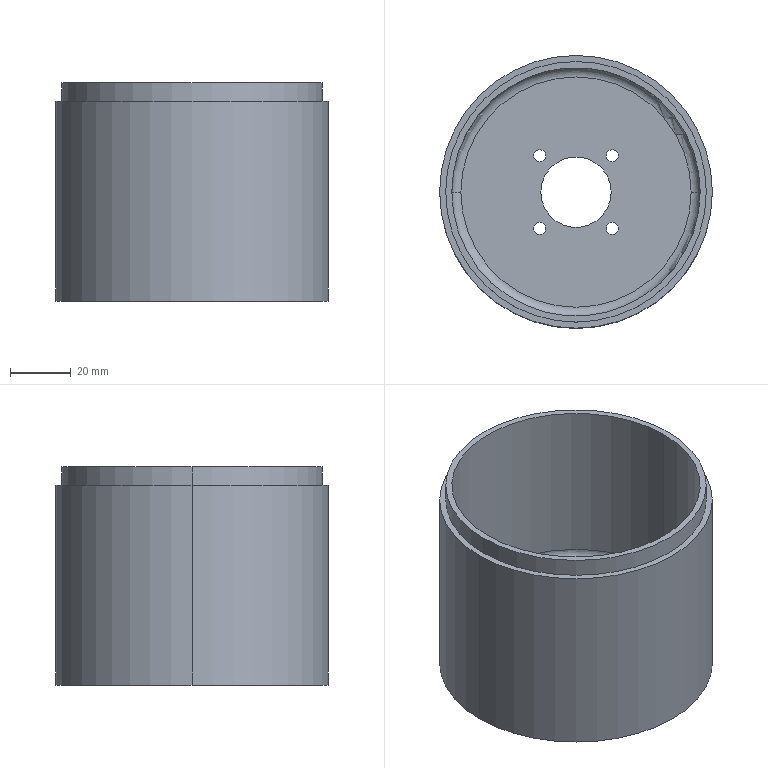Component | SolidWorks | g11-1 | 1 solid | 29 faces | box 90 x 90 x 72 mm | volume 87724 mm3 | cylinder 18 | plane 6 | torus 4 | sphere 1 | commonest cylinder face diameters 4 x8 86 x4 82 x4 90 x2
STEP:
#1=COLOUR_RGB('',0.7922,0.8196,0.9333);
#2=FILL_AREA_STYLE_COLOUR('',#1);
#3=FILL_AREA_STYLE('',(#2));
#4=SURFACE_STYLE_FILL_AREA(#3);
#5=SURFACE_SIDE_STYLE('',(#4));
#6=SURFACE_STYLE_USAGE(.BOTH.,#5);
#7=PRESENTATION_STYLE_ASSIGNMENT((#6));
#8=CARTESIAN_POINT('',(1.066,-0.06694,2.598));
#9=VERTEX_POINT('',#8);
#10=CARTESIAN_POINT('',(-2.32,-0.06694,2.598));
#11=VERTEX_POINT('',#10);
#12=CARTESIAN_POINT('',(-0.6271,-0.06694,2.598));
#13=DIRECTION('',(0.,0.,-1.));
#14=DIRECTION('',(-1.,0.,0.));
#15=AXIS2_PLACEMENT_3D('',#12,#13,#14);
#16=CIRCLE('',#15,1.693);
#17=EDGE_CURVE('',#9,#11,#16,.T.);
#18=ORIENTED_EDGE('',*,*,#17,.F.);
#19=CARTESIAN_POINT('',(1.066,-0.06694,2.441));
#20=VERTEX_POINT('',#19);
#21=CARTESIAN_POINT('',(1.066,-0.06694,2.165));
#22=DIRECTION('',(0.,0.,-1.));
#23=VECTOR('',#22,39.37);
#24=LINE('',#21,#23);
#25=EDGE_CURVE('',#9,#20,#24,.T.);
#26=ORIENTED_EDGE('',*,*,#25,.T.);
#27=CARTESIAN_POINT('',(-2.32,-0.06694,2.441));
#28=VERTEX_POINT('',#27);
#29=CARTESIAN_POINT('',(-0.6271,-0.06694,2.441));
#30=DIRECTION('',(0.,0.,-1.));
#31=DIRECTION('',(-1.,0.,0.));
#32=AXIS2_PLACEMENT_3D('',#29,#30,#31);
#33=CIRCLE('',#32,1.693);
#34=EDGE_CURVE('',#20,#28,#33,.T.);
#35=ORIENTED_EDGE('',*,*,#34,.T.);
#36=CARTESIAN_POINT('',(-2.32,-0.06694,2.165));
#37=DIRECTION('',(0.,0.,-1.));
#38=VECTOR('',#37,39.37);
#39=LINE('',#36,#38);
#40=EDGE_CURVE('',#11,#28,#39,.T.);
#41=ORIENTED_EDGE('',*,*,#40,.F.);
#42=EDGE_LOOP('',(#18,#26,#35,#41));
#43=FACE_OUTER_BOUND('',#42,.T.);
#44=CARTESIAN_POINT('',(-0.6271,-0.06694,2.165));
#45=DIRECTION('',(0.,0.,-1.));
#46=DIRECTION('',(-1.,0.,0.));
#47=AXIS2_PLACEMENT_3D('',#44,#45,#46);
#48=CYLINDRICAL_SURFACE('',#47,1.693);
#49=ADVANCED_FACE('',(#43),#48,.F.);
#50=CARTESIAN_POINT('',(-1.178,0.4055,2.992));
#51=VERTEX_POINT('',#50);
#52=CARTESIAN_POINT('',(-1.021,0.4055,2.992));
#53=VERTEX_POINT('',#52);
#54=CARTESIAN_POINT('',(-1.1,0.4055,2.992));
#55=DIRECTION('',(0.,0.,1.));
#56=DIRECTION('',(1.,0.,0.));
#57=AXIS2_PLACEMENT_3D('',#54,#55,#56);
#58=CIRCLE('',#57,0.07874);
#59=EDGE_CURVE('',#51,#53,#58,.T.);
#60=ORIENTED_EDGE('',*,*,#59,.T.);
#61=CARTESIAN_POINT('',(-1.021,0.4055,2.874));
#62=VERTEX_POINT('',#61);
#63=CARTESIAN_POINT('',(-1.021,0.4055,3.268));
#64=DIRECTION('',(0.,0.,-1.));
#65=VECTOR('',#64,39.37);
#66=LINE('',#63,#65);
#67=EDGE_CURVE('',#53,#62,#66,.T.);
#68=ORIENTED_EDGE('',*,*,#67,.T.);
#69=CARTESIAN_POINT('',(-1.178,0.4055,2.874));
#70=VERTEX_POINT('',#69);
#71=CARTESIAN_POINT('',(-1.1,0.4055,2.874));
#72=DIRECTION('',(0.,0.,-1.));
#73=DIRECTION('',(-1.,0.,0.));
#74=AXIS2_PLACEMENT_3D('',#71,#72,#73);
#75=CIRCLE('',#74,0.07874);
#76=EDGE_CURVE('',#62,#70,#75,.T.);
#77=ORIENTED_EDGE('',*,*,#76,.T.);
#78=CARTESIAN_POINT('',(-1.178,0.4055,3.268));
#79=DIRECTION('',(0.,0.,-1.));
#80=VECTOR('',#79,39.37);
#81=LINE('',#78,#80);
#82=EDGE_CURVE('',#51,#70,#81,.T.);
#83=ORIENTED_EDGE('',*,*,#82,.F.);
#84=EDGE_LOOP('',(#60,#68,#77,#83));
#85=FACE_OUTER_BOUND('',#84,.T.);
#86=CARTESIAN_POINT('',(-1.1,0.4055,3.268));
#87=DIRECTION('',(0.,0.,-1.));
#88=DIRECTION('',(-1.,0.,0.));
#89=AXIS2_PLACEMENT_3D('',#86,#87,#88);
#90=CYLINDRICAL_SURFACE('',#89,0.07874);
#91=ADVANCED_FACE('',(#85),#90,.F.);
#92=CARTESIAN_POINT('',(-0.2334,0.4055,2.992));
#93=VERTEX_POINT('',#92);
#94=CARTESIAN_POINT('',(-0.07591,0.4055,2.992));
#95=VERTEX_POINT('',#94);
#96=CARTESIAN_POINT('',(-0.1546,0.4055,2.992));
#97=DIRECTION('',(0.,0.,1.));
#98=DIRECTION('',(1.,0.,0.));
#99=AXIS2_PLACEMENT_3D('',#96,#97,#98);
#100=CIRCLE('',#99,0.07874);
#101=EDGE_CURVE('',#93,#95,#100,.T.);
#102=ORIENTED_EDGE('',*,*,#101,.T.);
#103=CARTESIAN_POINT('',(-0.07591,0.4055,2.874));
#104=VERTEX_POINT('',#103);
#105=CARTESIAN_POINT('',(-0.07591,0.4055,3.268));
#106=DIRECTION('',(0.,0.,-1.));
#107=VECTOR('',#106,39.37);
#108=LINE('',#105,#107);
#109=EDGE_CURVE('',#95,#104,#108,.T.);
#110=ORIENTED_EDGE('',*,*,#109,.T.);
#111=CARTESIAN_POINT('',(-0.2334,0.4055,2.874));
#112=VERTEX_POINT('',#111);
#113=CARTESIAN_POINT('',(-0.1546,0.4055,2.874));
#114=DIRECTION('',(0.,0.,-1.));
#115=DIRECTION('',(-1.,0.,0.));
#116=AXIS2_PLACEMENT_3D('',#113,#114,#115);
#117=CIRCLE('',#116,0.07874);
#118=EDGE_CURVE('',#104,#112,#117,.T.);
#119=ORIENTED_EDGE('',*,*,#118,.T.);
#120=CARTESIAN_POINT('',(-0.2334,0.4055,3.268));
#121=DIRECTION('',(0.,0.,-1.));
#122=VECTOR('',#121,39.37);
#123=LINE('',#120,#122);
#124=EDGE_CURVE('',#93,#112,#123,.T.);
#125=ORIENTED_EDGE('',*,*,#124,.F.);
#126=EDGE_LOOP('',(#102,#110,#119,#125));
#127=FACE_OUTER_BOUND('',#126,.T.);
#128=CARTESIAN_POINT('',(-0.1546,0.4055,3.268));
#129=DIRECTION('',(0.,0.,-1.));
#130=DIRECTION('',(-1.,0.,0.));
#131=AXIS2_PLACEMENT_3D('',#128,#129,#130);
#132=CYLINDRICAL_SURFACE('',#131,0.07874);
#133=ADVANCED_FACE('',(#127),#132,.F.);
#134=CARTESIAN_POINT('',(-0.2334,-0.5394,2.992));
#135=VERTEX_POINT('',#134);
#136=CARTESIAN_POINT('',(-0.07591,-0.5394,2.992));
#137=VERTEX_POINT('',#136);
#138=CARTESIAN_POINT('',(-0.1546,-0.5394,2.992));
#139=DIRECTION('',(0.,0.,1.));
#140=DIRECTION('',(1.,0.,0.));
#141=AXIS2_PLACEMENT_3D('',#138,#139,#140);
#142=CIRCLE('',#141,0.07874);
#143=EDGE_CURVE('',#135,#137,#142,.T.);
#144=ORIENTED_EDGE('',*,*,#143,.T.);
#145=CARTESIAN_POINT('',(-0.07591,-0.5394,2.874));
#146=VERTEX_POINT('',#145);
#147=CARTESIAN_POINT('',(-0.07591,-0.5394,3.268));
#148=DIRECTION('',(0.,0.,-1.));
#149=VECTOR('',#148,39.37);
#150=LINE('',#147,#149);
#151=EDGE_CURVE('',#137,#146,#150,.T.);
#152=ORIENTED_EDGE('',*,*,#151,.T.);
#153=CARTESIAN_POINT('',(-0.2334,-0.5394,2.874));
#154=VERTEX_POINT('',#153);
#155=CARTESIAN_POINT('',(-0.1546,-0.5394,2.874));
#156=DIRECTION('',(0.,0.,-1.));
#157=DIRECTION('',(-1.,0.,0.));
#158=AXIS2_PLACEMENT_3D('',#155,#156,#157);
#159=CIRCLE('',#158,0.07874);
#160=EDGE_CURVE('',#146,#154,#159,.T.);
#161=ORIENTED_EDGE('',*,*,#160,.T.);
#162=CARTESIAN_POINT('',(-0.2334,-0.5394,3.268));
#163=DIRECTION('',(0.,0.,-1.));
#164=VECTOR('',#163,39.37);
#165=LINE('',#162,#164);
#166=EDGE_CURVE('',#135,#154,#165,.T.);
#167=ORIENTED_EDGE('',*,*,#166,.F.);
#168=EDGE_LOOP('',(#144,#152,#161,#167));
#169=FACE_OUTER_BOUND('',#168,.T.);
#170=CARTESIAN_POINT('',(-0.1546,-0.5394,3.268));
#171=DIRECTION('',(0.,0.,-1.));
#172=DIRECTION('',(-1.,0.,0.));
#173=AXIS2_PLACEMENT_3D('',#170,#171,#172);
#174=CYLINDRICAL_SURFACE('',#173,0.07874);
#175=ADVANCED_FACE('',(#169),#174,.F.);
#176=CARTESIAN_POINT('',(-1.178,-0.5394,2.992));
#177=VERTEX_POINT('',#176);
#178=CARTESIAN_POINT('',(-1.021,-0.5394,2.992));
#179=VERTEX_POINT('',#178);
#180=CARTESIAN_POINT('',(-1.1,-0.5394,2.992));
#181=DIRECTION('',(0.,0.,1.));
#182=DIRECTION('',(1.,0.,0.));
#183=AXIS2_PLACEMENT_3D('',#180,#181,#182);
#184=CIRCLE('',#183,0.07874);
#185=EDGE_CURVE('',#177,#179,#184,.T.);
#186=ORIENTED_EDGE('',*,*,#185,.T.);
#187=CARTESIAN_POINT('',(-1.021,-0.5394,2.874));
#188=VERTEX_POINT('',#187);
#189=CARTESIAN_POINT('',(-1.021,-0.5394,3.268));
#190=DIRECTION('',(0.,0.,-1.));
#191=VECTOR('',#190,39.37);
#192=LINE('',#189,#191);
#193=EDGE_CURVE('',#179,#188,#192,.T.);
#194=ORIENTED_EDGE('',*,*,#193,.T.);
#195=CARTESIAN_POINT('',(-1.178,-0.5394,2.874));
#196=VERTEX_POINT('',#195);
#197=CARTESIAN_POINT('',(-1.1,-0.5394,2.874));
#198=DIRECTION('',(0.,0.,-1.));
#199=DIRECTION('',(-1.,0.,0.));
#200=AXIS2_PLACEMENT_3D('',#197,#198,#199);
#201=CIRCLE('',#200,0.07874);
#202=EDGE_CURVE('',#188,#196,#201,.T.);
#203=ORIENTED_EDGE('',*,*,#202,.T.);
#204=CARTESIAN_POINT('',(-1.178,-0.5394,3.268));
#205=DIRECTION('',(0.,0.,-1.));
#206=VECTOR('',#205,39.37);
#207=LINE('',#204,#206);
#208=EDGE_CURVE('',#177,#196,#207,.T.);
#209=ORIENTED_EDGE('',*,*,#208,.F.);
#210=EDGE_LOOP('',(#186,#194,#203,#209));
#211=FACE_OUTER_BOUND('',#210,.T.);
#212=CARTESIAN_POINT('',(-1.1,-0.5394,3.268));
#213=DIRECTION('',(0.,0.,-1.));
#214=DIRECTION('',(-1.,0.,0.));
#215=AXIS2_PLACEMENT_3D('',#212,#213,#214);
#216=CYLINDRICAL_SURFACE('',#215,0.07874);
#217=ADVANCED_FACE('',(#211),#216,.F.);
#218=CARTESIAN_POINT('',(0.869,-0.06694,2.874));
#219=VERTEX_POINT('',#218);
#220=CARTESIAN_POINT('',(-2.123,-0.06694,2.874));
#221=VERTEX_POINT('',#220);
#222=CARTESIAN_POINT('',(-0.6271,-0.06694,2.874));
#223=DIRECTION('',(0.,0.,-1.));
#224=DIRECTION('',(-1.,0.,0.));
#225=AXIS2_PLACEMENT_3D('',#222,#223,#224);
#226=CIRCLE('',#225,1.496);
#227=EDGE_CURVE('',#219,#221,#226,.T.);
#228=ORIENTED_EDGE('',*,*,#227,.F.);
#229=CARTESIAN_POINT('',(0.9871,-0.06694,2.756));
#230=VERTEX_POINT('',#229);
#231=CARTESIAN_POINT('',(0.869,-0.06694,2.756));
#232=DIRECTION('',(-0.,1.,0.));
#233=DIRECTION('',(-1.,-0.,0.));
#234=AXIS2_PLACEMENT_3D('',#231,#232,#233);
#235=CIRCLE('',#234,0.1181);
#236=EDGE_CURVE('',#219,#230,#235,.T.);
#237=ORIENTED_EDGE('',*,*,#236,.T.);
#238=CARTESIAN_POINT('',(-2.241,-0.06694,2.756));
#239=VERTEX_POINT('',#238);
#240=CARTESIAN_POINT('',(-0.6271,-0.06694,2.756));
#241=DIRECTION('',(0.,0.,1.));
#242=DIRECTION('',(-1.,0.,0.));
#243=AXIS2_PLACEMENT_3D('',#240,#241,#242);
#244=CIRCLE('',#243,1.614);
#245=EDGE_CURVE('',#239,#230,#244,.T.);
#246=ORIENTED_EDGE('',*,*,#245,.F.);
#247=CARTESIAN_POINT('',(-2.123,-0.06694,2.756));
#248=DIRECTION('',(0.,-1.,0.));
#249=DIRECTION('',(0.,0.,-1.));
#250=AXIS2_PLACEMENT_3D('',#247,#248,#249);
#251=CIRCLE('',#250,0.1181);
#252=EDGE_CURVE('',#221,#239,#251,.T.);
#253=ORIENTED_EDGE('',*,*,#252,.F.);
#254=EDGE_LOOP('',(#228,#237,#246,#253));
#255=FACE_OUTER_BOUND('',#254,.T.);
#256=CARTESIAN_POINT('',(-0.6271,-0.06694,2.756));
#257=DIRECTION('',(0.,0.,-1.));
#258=DIRECTION('',(-1.,0.,0.));
#259=AXIS2_PLACEMENT_3D('',#256,#257,#258);
#260=TOROIDAL_SURFACE('',#259,1.496,0.1181);
#261=ADVANCED_FACE('',(#255),#260,.F.);
#262=CARTESIAN_POINT('',(-2.123,-0.06694,2.992));
#263=VERTEX_POINT('',#262);
#264=CARTESIAN_POINT('',(0.869,-0.06694,2.992));
#265=VERTEX_POINT('',#264);
#266=CARTESIAN_POINT('',(-0.6271,-0.06694,2.992));
#267=DIRECTION('',(0.,0.,1.));
#268=DIRECTION('',(1.,0.,0.));
#269=AXIS2_PLACEMENT_3D('',#266,#267,#268);
#270=CIRCLE('',#269,1.496);
#271=EDGE_CURVE('',#263,#265,#270,.T.);
#272=ORIENTED_EDGE('',*,*,#271,.F.);
#273=CARTESIAN_POINT('',(-2.241,-0.06694,3.11));
#274=VERTEX_POINT('',#273);
#275=CARTESIAN_POINT('',(-2.123,-0.06694,3.11));
#276=DIRECTION('',(0.,1.,0.));
#277=DIRECTION('',(-1.,0.,0.));
#278=AXIS2_PLACEMENT_3D('',#275,#276,#277);
#279=CIRCLE('',#278,0.1181);
#280=EDGE_CURVE('',#263,#274,#279,.T.);
#281=ORIENTED_EDGE('',*,*,#280,.T.);
#282=CARTESIAN_POINT('',(0.9871,-0.06694,3.11));
#283=VERTEX_POINT('',#282);
#284=CARTESIAN_POINT('',(-0.6271,-0.06694,3.11));
#285=DIRECTION('',(0.,0.,-1.));
#286=DIRECTION('',(1.,0.,0.));
#287=AXIS2_PLACEMENT_3D('',#284,#285,#286);
#288=CIRCLE('',#287,1.614);
#289=EDGE_CURVE('',#283,#274,#288,.T.);
#290=ORIENTED_EDGE('',*,*,#289,.F.);
#291=CARTESIAN_POINT('',(0.869,-0.06694,3.11));
#292=DIRECTION('',(0.,-1.,0.));
#293=DIRECTION('',(0.,0.,-1.));
#294=AXIS2_PLACEMENT_3D('',#291,#292,#293);
#295=CIRCLE('',#294,0.1181);
#296=EDGE_CURVE('',#265,#283,#295,.T.);
#297=ORIENTED_EDGE('',*,*,#296,.F.);
#298=EDGE_LOOP('',(#272,#281,#290,#297));
#299=FACE_OUTER_BOUND('',#298,.T.);
#300=CARTESIAN_POINT('',(-0.6271,-0.06694,3.11));
#301=DIRECTION('',(0.,0.,1.));
#302=DIRECTION('',(1.,0.,0.));
#303=AXIS2_PLACEMENT_3D('',#300,#301,#302);
#304=TOROIDAL_SURFACE('',#303,1.496,0.1181);
#305=ADVANCED_FACE('',(#299),#304,.F.);
#306=CARTESIAN_POINT('',(-2.32,-0.06694,5.276));
#307=VERTEX_POINT('',#306);
#308=CARTESIAN_POINT('',(1.066,-0.06694,5.276));
#309=VERTEX_POINT('',#308);
#310=CARTESIAN_POINT('',(-0.6271,-0.06694,5.276));
#311=DIRECTION('',(0.,0.,-1.));
#312=DIRECTION('',(-1.,0.,0.));
#313=AXIS2_PLACEMENT_3D('',#310,#311,#312);
#314=CIRCLE('',#313,1.693);
#315=EDGE_CURVE('',#307,#309,#314,.T.);
#316=ORIENTED_EDGE('',*,*,#315,.T.);
#317=CARTESIAN_POINT('',(1.066,-0.06694,5.039));
#318=VERTEX_POINT('',#317);
#319=CARTESIAN_POINT('',(1.066,-0.06694,5.276));
#320=DIRECTION('',(0.,0.,-1.));
#321=VECTOR('',#320,39.37);
#322=LINE('',#319,#321);
#323=EDGE_CURVE('',#309,#318,#322,.T.);
#324=ORIENTED_EDGE('',*,*,#323,.T.);
#325=CARTESIAN_POINT('',(-2.32,-0.06694,5.039));
#326=VERTEX_POINT('',#325);
#327=CARTESIAN_POINT('',(-0.6271,-0.06694,5.039));
#328=DIRECTION('',(0.,0.,1.));
#329=DIRECTION('',(1.,0.,0.));
#330=AXIS2_PLACEMENT_3D('',#327,#328,#329);
#331=CIRCLE('',#330,1.693);
#332=EDGE_CURVE('',#318,#326,#331,.T.);
#333=ORIENTED_EDGE('',*,*,#332,.T.);
#334=CARTESIAN_POINT('',(-2.32,-0.06694,5.276));
#335=DIRECTION('',(0.,0.,-1.));
#336=VECTOR('',#335,39.37);
#337=LINE('',#334,#336);
#338=EDGE_CURVE('',#307,#326,#337,.T.);
#339=ORIENTED_EDGE('',*,*,#338,.F.);
#340=EDGE_LOOP('',(#316,#324,#333,#339));
#341=FACE_OUTER_BOUND('',#340,.T.);
#342=CARTESIAN_POINT('',(-0.6271,-0.06694,5.276));
#343=DIRECTION('',(0.,0.,-1.));
#344=DIRECTION('',(-1.,0.,0.));
#345=AXIS2_PLACEMENT_3D('',#342,#343,#344);
#346=CYLINDRICAL_SURFACE('',#345,1.693);
#347=ADVANCED_FACE('',(#341),#346,.T.);
#348=ORIENTED_EDGE('',*,*,#245,.T.);
#349=CARTESIAN_POINT('',(0.9871,-0.06694,2.598));
#350=VERTEX_POINT('',#349);
#351=CARTESIAN_POINT('',(0.9871,-0.06694,5.039));
#352=DIRECTION('',(0.,0.,-1.));
#353=VECTOR('',#352,39.37);
#354=LINE('',#351,#353);
#355=EDGE_CURVE('',#230,#350,#354,.T.);
#356=ORIENTED_EDGE('',*,*,#355,.T.);
#357=CARTESIAN_POINT('',(-2.241,-0.06694,2.598));
#358=VERTEX_POINT('',#357);
#359=CARTESIAN_POINT('',(-0.6271,-0.06694,2.598));
#360=DIRECTION('',(0.,0.,1.));
#361=DIRECTION('',(1.,0.,0.));
#362=AXIS2_PLACEMENT_3D('',#359,#360,#361);
#363=CIRCLE('',#362,1.614);
#364=EDGE_CURVE('',#358,#350,#363,.T.);
#365=ORIENTED_EDGE('',*,*,#364,.F.);
#366=CARTESIAN_POINT('',(-2.241,-0.06694,5.039));
#367=DIRECTION('',(0.,0.,-1.));
#368=VECTOR('',#367,39.37);
#369=LINE('',#366,#368);
#370=EDGE_CURVE('',#239,#358,#369,.T.);
#371=ORIENTED_EDGE('',*,*,#370,.F.);
#372=EDGE_LOOP('',(#348,#356,#365,#371));
#373=FACE_OUTER_BOUND('',#372,.T.);
#374=CARTESIAN_POINT('',(-0.6271,-0.06694,5.039));
#375=DIRECTION('',(0.,0.,-1.));
#376=DIRECTION('',(-1.,0.,0.));
#377=AXIS2_PLACEMENT_3D('',#374,#375,#376);
#378=CYLINDRICAL_SURFACE('',#377,1.614);
#379=ADVANCED_FACE('',(#373),#378,.F.);
#380=CARTESIAN_POINT('',(1.145,-0.06694,5.039));
#381=VERTEX_POINT('',#380);
#382=CARTESIAN_POINT('',(-2.399,-0.06694,5.039));
#383=VERTEX_POINT('',#382);
#384=CARTESIAN_POINT('',(-0.6271,-0.06694,5.039));
#385=DIRECTION('',(0.,0.,1.));
#386=DIRECTION('',(1.,0.,0.));
#387=AXIS2_PLACEMENT_3D('',#384,#385,#386);
#388=CIRCLE('',#387,1.772);
#389=EDGE_CURVE('',#381,#383,#388,.T.);
#390=ORIENTED_EDGE('',*,*,#389,.F.);
#391=CARTESIAN_POINT('',(1.145,-0.06694,2.441));
#392=VERTEX_POINT('',#391);
#393=CARTESIAN_POINT('',(1.145,-0.06694,5.039));
#394=DIRECTION('',(0.,0.,-1.));
#395=VECTOR('',#394,39.37);
#396=LINE('',#393,#395);
#397=EDGE_CURVE('',#381,#392,#396,.T.);
#398=ORIENTED_EDGE('',*,*,#397,.T.);
#399=CARTESIAN_POINT('',(-2.399,-0.06694,2.441));
#400=VERTEX_POINT('',#399);
#401=CARTESIAN_POINT('',(-0.6271,-0.06694,2.441));
#402=DIRECTION('',(0.,0.,-1.));
#403=DIRECTION('',(-1.,0.,0.));
#404=AXIS2_PLACEMENT_3D('',#401,#402,#403);
#405=CIRCLE('',#404,1.772);
#406=EDGE_CURVE('',#400,#392,#405,.T.);
#407=ORIENTED_EDGE('',*,*,#406,.F.);
#408=CARTESIAN_POINT('',(-2.399,-0.06694,5.039));
#409=DIRECTION('',(0.,0.,-1.));
#410=VECTOR('',#409,39.37);
#411=LINE('',#408,#410);
#412=EDGE_CURVE('',#383,#400,#411,.T.);
#413=ORIENTED_EDGE('',*,*,#412,.F.);
#414=EDGE_LOOP('',(#390,#398,#407,#413));
#415=FACE_OUTER_BOUND('',#414,.T.);
#416=CARTESIAN_POINT('',(-0.6271,-0.06694,5.039));
#417=DIRECTION('',(0.,0.,-1.));
#418=DIRECTION('',(-1.,0.,0.));
#419=AXIS2_PLACEMENT_3D('',#416,#417,#418);
#420=CYLINDRICAL_SURFACE('',#419,1.772);
#421=ADVANCED_FACE('',(#415),#420,.T.);
#422=CARTESIAN_POINT('',(0.9871,-0.06694,5.276));
#423=VERTEX_POINT('',#422);
#424=CARTESIAN_POINT('',(-2.241,-0.06694,5.276));
#425=VERTEX_POINT('',#424);
#426=CARTESIAN_POINT('',(-0.6271,-0.06694,5.276));
#427=DIRECTION('',(0.,0.,-1.));
#428=DIRECTION('',(-1.,0.,0.));
#429=AXIS2_PLACEMENT_3D('',#426,#427,#428);
#430=CIRCLE('',#429,1.614);
#431=EDGE_CURVE('',#423,#425,#430,.T.);
#432=ORIENTED_EDGE('',*,*,#431,.F.);
#433=CARTESIAN_POINT('',(0.9871,-0.06694,5.039));
#434=DIRECTION('',(0.,0.,-1.));
#435=VECTOR('',#434,39.37);
#436=LINE('',#433,#435);
#437=EDGE_CURVE('',#423,#283,#436,.T.);
#438=ORIENTED_EDGE('',*,*,#437,.T.);
#439=ORIENTED_EDGE('',*,*,#289,.T.);
#440=CARTESIAN_POINT('',(-2.241,-0.06694,5.039));
#441=DIRECTION('',(0.,0.,-1.));
#442=VECTOR('',#441,39.37);
#443=LINE('',#440,#442);
#444=EDGE_CURVE('',#425,#274,#443,.T.);
#445=ORIENTED_EDGE('',*,*,#444,.F.);
#446=EDGE_LOOP('',(#432,#438,#439,#445));
#447=FACE_OUTER_BOUND('',#446,.T.);
#448=CARTESIAN_POINT('',(-0.6271,-0.06694,5.039));
#449=DIRECTION('',(0.,0.,-1.));
#450=DIRECTION('',(-1.,0.,0.));
#451=AXIS2_PLACEMENT_3D('',#448,#449,#450);
#452=CYLINDRICAL_SURFACE('',#451,1.614);
#453=ADVANCED_FACE('',(#447),#452,.F.);
#454=ORIENTED_EDGE('',*,*,#437,.F.);
#455=CARTESIAN_POINT('',(-0.6271,-0.06694,5.276));
#456=DIRECTION('',(0.,0.,-1.));
#457=DIRECTION('',(-1.,0.,0.));
#458=AXIS2_PLACEMENT_3D('',#455,#456,#457);
#459=CIRCLE('',#458,1.614);
#460=EDGE_CURVE('',#425,#423,#459,.T.);
#461=ORIENTED_EDGE('',*,*,#460,.F.);
#462=ORIENTED_EDGE('',*,*,#444,.T.);
#463=CARTESIAN_POINT('',(-0.6271,-0.06694,3.11));
#464=DIRECTION('',(0.,0.,-1.));
#465=DIRECTION('',(1.,0.,0.));
#466=AXIS2_PLACEMENT_3D('',#463,#464,#465);
#467=CIRCLE('',#466,1.614);
#468=EDGE_CURVE('',#274,#283,#467,.T.);
#469=ORIENTED_EDGE('',*,*,#468,.T.);
#470=EDGE_LOOP('',(#454,#461,#462,#469));
#471=FACE_OUTER_BOUND('',#470,.T.);
#472=CARTESIAN_POINT('',(-0.6271,-0.06694,5.039));
#473=DIRECTION('',(0.,0.,-1.));
#474=DIRECTION('',(-1.,0.,0.));
#475=AXIS2_PLACEMENT_3D('',#472,#473,#474);
#476=CYLINDRICAL_SURFACE('',#475,1.614);
#477=ADVANCED_FACE('',(#471),#476,.F.);
#478=CARTESIAN_POINT('',(-0.6271,-0.06694,5.039));
#479=DIRECTION('',(0.,0.,1.));
#480=DIRECTION('',(1.,0.,0.));
#481=AXIS2_PLACEMENT_3D('',#478,#479,#480);
#482=CIRCLE('',#481,1.693);
#483=EDGE_CURVE('',#326,#318,#482,.T.);
#484=ORIENTED_EDGE('',*,*,#483,.F.);
#485=ORIENTED_EDGE('',*,*,#332,.F.);
#486=EDGE_LOOP('',(#484,#485));
#487=FACE_BOUND('',#486,.T.);
#488=CARTESIAN_POINT('',(-0.6271,-0.06694,5.039));
#489=DIRECTION('',(0.,0.,1.));
#490=DIRECTION('',(1.,0.,0.));
#491=AXIS2_PLACEMENT_3D('',#488,#489,#490);
#492=CIRCLE('',#491,1.772);
#493=EDGE_CURVE('',#383,#381,#492,.T.);
#494=ORIENTED_EDGE('',*,*,#493,.T.);
#495=ORIENTED_EDGE('',*,*,#389,.T.);
#496=EDGE_LOOP('',(#494,#495));
#497=FACE_OUTER_BOUND('',#496,.T.);
#498=CARTESIAN_POINT('',(-0.6271,-0.06694,5.039));
#499=DIRECTION('',(0.,0.,1.));
#500=DIRECTION('',(1.,0.,0.));
#501=AXIS2_PLACEMENT_3D('',#498,#499,#500);
#502=PLANE('',#501);
#503=ADVANCED_FACE('',(#487,#497),#502,.T.);
#504=ORIENTED_EDGE('',*,*,#397,.F.);
#505=ORIENTED_EDGE('',*,*,#493,.F.);
#506=ORIENTED_EDGE('',*,*,#412,.T.);
#507=CARTESIAN_POINT('',(-0.6271,-0.06694,2.441));
#508=DIRECTION('',(0.,0.,-1.));
#509=DIRECTION('',(-1.,0.,0.));
#510=AXIS2_PLACEMENT_3D('',#507,#508,#509);
#511=CIRCLE('',#510,1.772);
#512=EDGE_CURVE('',#392,#400,#511,.T.);
#513=ORIENTED_EDGE('',*,*,#512,.F.);
#514=EDGE_LOOP('',(#504,#505,#506,#513));
#515=FACE_OUTER_BOUND('',#514,.T.);
#516=CARTESIAN_POINT('',(-0.6271,-0.06694,5.039));
#517=DIRECTION('',(0.,0.,-1.));
#518=DIRECTION('',(-1.,0.,0.));
#519=AXIS2_PLACEMENT_3D('',#516,#517,#518);
#520=CYLINDRICAL_SURFACE('',#519,1.772);
#521=ADVANCED_FACE('',(#515),#520,.T.);
#522=ORIENTED_EDGE('',*,*,#355,.F.);
#523=CARTESIAN_POINT('',(-0.6271,-0.06694,2.756));
#524=DIRECTION('',(0.,0.,1.));
#525=DIRECTION('',(-1.,0.,0.));
#526=AXIS2_PLACEMENT_3D('',#523,#524,#525);
#527=CIRCLE('',#526,1.614);
#528=EDGE_CURVE('',#230,#239,#527,.T.);
#529=ORIENTED_EDGE('',*,*,#528,.T.);
#530=ORIENTED_EDGE('',*,*,#370,.T.);
#531=CARTESIAN_POINT('',(-0.6271,-0.06694,2.598));
#532=DIRECTION('',(0.,0.,1.));
#533=DIRECTION('',(1.,0.,0.));
#534=AXIS2_PLACEMENT_3D('',#531,#532,#533);
#535=CIRCLE('',#534,1.614);
#536=EDGE_CURVE('',#350,#358,#535,.T.);
#537=ORIENTED_EDGE('',*,*,#536,.F.);
#538=EDGE_LOOP('',(#522,#529,#530,#537));
#539=FACE_OUTER_BOUND('',#538,.T.);
#540=CARTESIAN_POINT('',(-0.6271,-0.06694,5.039));
#541=DIRECTION('',(0.,0.,-1.));
#542=DIRECTION('',(-1.,0.,0.));
#543=AXIS2_PLACEMENT_3D('',#540,#541,#542);
#544=CYLINDRICAL_SURFACE('',#543,1.614);
#545=ADVANCED_FACE('',(#539),#544,.F.);
#546=CARTESIAN_POINT('',(-0.6271,-0.06694,2.441));
#547=DIRECTION('',(0.,0.,-1.));
#548=DIRECTION('',(-1.,0.,0.));
#549=AXIS2_PLACEMENT_3D('',#546,#547,#548);
#550=CIRCLE('',#549,1.693);
#551=EDGE_CURVE('',#28,#20,#550,.T.);
#552=ORIENTED_EDGE('',*,*,#551,.F.);
#553=ORIENTED_EDGE('',*,*,#34,.F.);
#554=EDGE_LOOP('',(#552,#553));
#555=FACE_BOUND('',#554,.T.);
#556=ORIENTED_EDGE('',*,*,#406,.T.);
#557=ORIENTED_EDGE('',*,*,#512,.T.);
#558=EDGE_LOOP('',(#556,#557));
#559=FACE_OUTER_BOUND('',#558,.T.);
#560=CARTESIAN_POINT('',(-0.6271,-0.06694,2.441));
#561=DIRECTION('',(0.,0.,-1.));
#562=DIRECTION('',(-1.,0.,0.));
#563=AXIS2_PLACEMENT_3D('',#560,#561,#562);
#564=PLANE('',#563);
#565=ADVANCED_FACE('',(#555,#559),#564,.T.);
#566=ORIENTED_EDGE('',*,*,#323,.F.);
#567=CARTESIAN_POINT('',(-0.6271,-0.06694,5.276));
#568=DIRECTION('',(0.,0.,-1.));
#569=DIRECTION('',(-1.,0.,0.));
#570=AXIS2_PLACEMENT_3D('',#567,#568,#569);
#571=CIRCLE('',#570,1.693);
#572=EDGE_CURVE('',#309,#307,#571,.T.);
#573=ORIENTED_EDGE('',*,*,#572,.T.);
#574=ORIENTED_EDGE('',*,*,#338,.T.);
#575=ORIENTED_EDGE('',*,*,#483,.T.);
#576=EDGE_LOOP('',(#566,#573,#574,#575));
#577=FACE_OUTER_BOUND('',#576,.T.);
#578=CARTESIAN_POINT('',(-0.6271,-0.06694,5.276));
#579=DIRECTION('',(0.,0.,-1.));
#580=DIRECTION('',(-1.,0.,0.));
#581=AXIS2_PLACEMENT_3D('',#578,#579,#580);
#582=CYLINDRICAL_SURFACE('',#581,1.693);
#583=ADVANCED_FACE('',(#577),#582,.T.);
#584=ORIENTED_EDGE('',*,*,#460,.T.);
#585=ORIENTED_EDGE('',*,*,#431,.T.);
#586=EDGE_LOOP('',(#584,#585));
#587=FACE_BOUND('',#586,.T.);
#588=ORIENTED_EDGE('',*,*,#315,.F.);
#589=ORIENTED_EDGE('',*,*,#572,.F.);
#590=EDGE_LOOP('',(#588,#589));
#591=FACE_OUTER_BOUND('',#590,.T.);
#592=CARTESIAN_POINT('',(-0.6271,-0.06694,5.276));
#593=DIRECTION('',(0.,0.,1.));
#594=DIRECTION('',(-1.,0.,0.));
#595=AXIS2_PLACEMENT_3D('',#592,#593,#594);
#596=PLANE('',#595);
#597=ADVANCED_FACE('',(#587,#591),#596,.T.);
#598=CARTESIAN_POINT('',(-0.1696,-0.06694,2.992));
#599=VERTEX_POINT('',#598);
#600=CARTESIAN_POINT('',(-1.085,-0.06694,2.992));
#601=VERTEX_POINT('',#600);
#602=CARTESIAN_POINT('',(-0.6271,-0.06694,2.992));
#603=DIRECTION('',(0.,0.,-1.));
#604=DIRECTION('',(1.,0.,0.));
#605=AXIS2_PLACEMENT_3D('',#602,#603,#604);
#606=CIRCLE('',#605,0.4574);
#607=EDGE_CURVE('',#599,#601,#606,.T.);
#608=ORIENTED_EDGE('',*,*,#607,.T.);
#609=CARTESIAN_POINT('',(-0.6271,-0.06694,2.992));
#610=DIRECTION('',(0.,0.,-1.));
#611=DIRECTION('',(1.,0.,0.));
#612=AXIS2_PLACEMENT_3D('',#609,#610,#611);
#613=CIRCLE('',#612,0.4574);
#614=EDGE_CURVE('',#601,#599,#613,.T.);
#615=ORIENTED_EDGE('',*,*,#614,.T.);
#616=EDGE_LOOP('',(#608,#615));
#617=FACE_BOUND('',#616,.T.);
#618=ORIENTED_EDGE('',*,*,#59,.F.);
#619=CARTESIAN_POINT('',(-1.1,0.4055,2.992));
#620=DIRECTION('',(0.,0.,1.));
#621=DIRECTION('',(1.,0.,0.));
#622=AXIS2_PLACEMENT_3D('',#619,#620,#621);
#623=CIRCLE('',#622,0.07874);
#624=EDGE_CURVE('',#53,#51,#623,.T.);
#625=ORIENTED_EDGE('',*,*,#624,.F.);
#626=EDGE_LOOP('',(#618,#625));
#627=FACE_BOUND('',#626,.T.);
#628=ORIENTED_EDGE('',*,*,#101,.F.);
#629=CARTESIAN_POINT('',(-0.1546,0.4055,2.992));
#630=DIRECTION('',(0.,0.,1.));
#631=DIRECTION('',(1.,0.,0.));
#632=AXIS2_PLACEMENT_3D('',#629,#630,#631);
#633=CIRCLE('',#632,0.07874);
#634=EDGE_CURVE('',#95,#93,#633,.T.);
#635=ORIENTED_EDGE('',*,*,#634,.F.);
#636=EDGE_LOOP('',(#628,#635));
#637=FACE_BOUND('',#636,.T.);
#638=ORIENTED_EDGE('',*,*,#143,.F.);
#639=CARTESIAN_POINT('',(-0.1546,-0.5394,2.992));
#640=DIRECTION('',(0.,0.,1.));
#641=DIRECTION('',(1.,0.,0.));
#642=AXIS2_PLACEMENT_3D('',#639,#640,#641);
#643=CIRCLE('',#642,0.07874);
#644=EDGE_CURVE('',#137,#135,#643,.T.);
#645=ORIENTED_EDGE('',*,*,#644,.F.);
#646=EDGE_LOOP('',(#638,#645));
#647=FACE_BOUND('',#646,.T.);
#648=ORIENTED_EDGE('',*,*,#185,.F.);
#649=CARTESIAN_POINT('',(-1.1,-0.5394,2.992));
#650=DIRECTION('',(0.,0.,1.));
#651=DIRECTION('',(1.,0.,0.));
#652=AXIS2_PLACEMENT_3D('',#649,#650,#651);
#653=CIRCLE('',#652,0.07874);
#654=EDGE_CURVE('',#179,#177,#653,.T.);
#655=ORIENTED_EDGE('',*,*,#654,.F.);
#656=EDGE_LOOP('',(#648,#655));
#657=FACE_BOUND('',#656,.T.);
#658=CARTESIAN_POINT('',(-0.6271,-0.06694,2.992));
#659=DIRECTION('',(0.,0.,1.));
#660=DIRECTION('',(1.,0.,0.));
#661=AXIS2_PLACEMENT_3D('',#658,#659,#660);
#662=CIRCLE('',#661,1.496);
#663=EDGE_CURVE('',#265,#263,#662,.T.);
#664=ORIENTED_EDGE('',*,*,#663,.T.);
#665=ORIENTED_EDGE('',*,*,#271,.T.);
#666=EDGE_LOOP('',(#664,#665));
#667=FACE_OUTER_BOUND('',#666,.T.);
#668=CARTESIAN_POINT('',(-2.399,-0.06694,2.992));
#669=DIRECTION('',(0.,0.,1.));
#670=DIRECTION('',(1.,0.,0.));
#671=AXIS2_PLACEMENT_3D('',#668,#669,#670);
#672=PLANE('',#671);
#673=ADVANCED_FACE('',(#617,#627,#637,#647,#657,#667),#672,.T.);
#674=CARTESIAN_POINT('',(-1.1,-0.06694,2.874));
#675=VERTEX_POINT('',#674);
#676=CARTESIAN_POINT('',(-0.1546,-0.06694,2.874));
#677=VERTEX_POINT('',#676);
#678=CARTESIAN_POINT('',(-0.6271,-0.06694,2.874));
#679=DIRECTION('',(0.,0.,1.));
#680=DIRECTION('',(-1.,0.,0.));
#681=AXIS2_PLACEMENT_3D('',#678,#679,#680);
#682=CIRCLE('',#681,0.4724);
#683=EDGE_CURVE('',#675,#677,#682,.T.);
#684=ORIENTED_EDGE('',*,*,#683,.T.);
#685=CARTESIAN_POINT('',(-0.6271,-0.06694,2.874));
#686=DIRECTION('',(0.,0.,1.));
#687=DIRECTION('',(-1.,0.,0.));
#688=AXIS2_PLACEMENT_3D('',#685,#686,#687);
#689=CIRCLE('',#688,0.4724);
#690=EDGE_CURVE('',#677,#675,#689,.T.);
#691=ORIENTED_EDGE('',*,*,#690,.T.);
#692=EDGE_LOOP('',(#684,#691));
#693=FACE_BOUND('',#692,.T.);
#694=CARTESIAN_POINT('',(-1.1,0.4055,2.874));
#695=DIRECTION('',(0.,0.,-1.));
#696=DIRECTION('',(-1.,0.,0.));
#697=AXIS2_PLACEMENT_3D('',#694,#695,#696);
#698=CIRCLE('',#697,0.07874);
#699=EDGE_CURVE('',#70,#62,#698,.T.);
#700=ORIENTED_EDGE('',*,*,#699,.F.);
#701=ORIENTED_EDGE('',*,*,#76,.F.);
#702=EDGE_LOOP('',(#700,#701));
#703=FACE_BOUND('',#702,.T.);
#704=CARTESIAN_POINT('',(-0.1546,0.4055,2.874));
#705=DIRECTION('',(0.,0.,-1.));
#706=DIRECTION('',(-1.,0.,0.));
#707=AXIS2_PLACEMENT_3D('',#704,#705,#706);
#708=CIRCLE('',#707,0.07874);
#709=EDGE_CURVE('',#112,#104,#708,.T.);
#710=ORIENTED_EDGE('',*,*,#709,.F.);
#711=ORIENTED_EDGE('',*,*,#118,.F.);
#712=EDGE_LOOP('',(#710,#711));
#713=FACE_BOUND('',#712,.T.);
#714=CARTESIAN_POINT('',(-0.1546,-0.5394,2.874));
#715=DIRECTION('',(0.,0.,-1.));
#716=DIRECTION('',(-1.,0.,0.));
#717=AXIS2_PLACEMENT_3D('',#714,#715,#716);
#718=CIRCLE('',#717,0.07874);
#719=EDGE_CURVE('',#154,#146,#718,.T.);
#720=ORIENTED_EDGE('',*,*,#719,.F.);
#721=ORIENTED_EDGE('',*,*,#160,.F.);
#722=EDGE_LOOP('',(#720,#721));
#723=FACE_BOUND('',#722,.T.);
#724=CARTESIAN_POINT('',(-1.1,-0.5394,2.874));
#725=DIRECTION('',(0.,0.,-1.));
#726=DIRECTION('',(-1.,0.,0.));
#727=AXIS2_PLACEMENT_3D('',#724,#725,#726);
#728=CIRCLE('',#727,0.07874);
#729=EDGE_CURVE('',#196,#188,#728,.T.);
#730=ORIENTED_EDGE('',*,*,#729,.F.);
#731=ORIENTED_EDGE('',*,*,#202,.F.);
#732=EDGE_LOOP('',(#730,#731));
#733=FACE_BOUND('',#732,.T.);
#734=CARTESIAN_POINT('',(-0.6271,-0.06694,2.874));
#735=DIRECTION('',(0.,0.,-1.));
#736=DIRECTION('',(-1.,0.,0.));
#737=AXIS2_PLACEMENT_3D('',#734,#735,#736);
#738=CIRCLE('',#737,1.496);
#739=EDGE_CURVE('',#221,#219,#738,.T.);
#740=ORIENTED_EDGE('',*,*,#739,.T.);
#741=ORIENTED_EDGE('',*,*,#227,.T.);
#742=EDGE_LOOP('',(#740,#741));
#743=FACE_OUTER_BOUND('',#742,.T.);
#744=CARTESIAN_POINT('',(-2.399,-0.06694,2.874));
#745=DIRECTION('',(0.,0.,-1.));
#746=DIRECTION('',(-1.,0.,0.));
#747=AXIS2_PLACEMENT_3D('',#744,#745,#746);
#748=PLANE('',#747);
#749=ADVANCED_FACE('',(#693,#703,#713,#723,#733,#743),#748,.T.);
#750=ORIENTED_EDGE('',*,*,#280,.F.);
#751=ORIENTED_EDGE('',*,*,#663,.F.);
#752=ORIENTED_EDGE('',*,*,#296,.T.);
#753=ORIENTED_EDGE('',*,*,#468,.F.);
#754=EDGE_LOOP('',(#750,#751,#752,#753));
#755=FACE_OUTER_BOUND('',#754,.T.);
#756=CARTESIAN_POINT('',(-0.6271,-0.06694,3.11));
#757=DIRECTION('',(0.,0.,1.));
#758=DIRECTION('',(1.,0.,0.));
#759=AXIS2_PLACEMENT_3D('',#756,#757,#758);
#760=TOROIDAL_SURFACE('',#759,1.496,0.1181);
#761=ADVANCED_FACE('',(#755),#760,.F.);
#762=ORIENTED_EDGE('',*,*,#236,.F.);
#763=ORIENTED_EDGE('',*,*,#739,.F.);
#764=ORIENTED_EDGE('',*,*,#252,.T.);
#765=ORIENTED_EDGE('',*,*,#528,.F.);
#766=EDGE_LOOP('',(#762,#763,#764,#765));
#767=FACE_OUTER_BOUND('',#766,.T.);
#768=CARTESIAN_POINT('',(-0.6271,-0.06694,2.756));
#769=DIRECTION('',(0.,0.,-1.));
#770=DIRECTION('',(-1.,0.,0.));
#771=AXIS2_PLACEMENT_3D('',#768,#769,#770);
#772=TOROIDAL_SURFACE('',#771,1.496,0.1181);
#773=ADVANCED_FACE('',(#767),#772,.F.);
#774=ORIENTED_EDGE('',*,*,#193,.F.);
#775=ORIENTED_EDGE('',*,*,#654,.T.);
#776=ORIENTED_EDGE('',*,*,#208,.T.);
#777=ORIENTED_EDGE('',*,*,#729,.T.);
#778=EDGE_LOOP('',(#774,#775,#776,#777));
#779=FACE_OUTER_BOUND('',#778,.T.);
#780=CARTESIAN_POINT('',(-1.1,-0.5394,3.268));
#781=DIRECTION('',(0.,0.,-1.));
#782=DIRECTION('',(-1.,0.,0.));
#783=AXIS2_PLACEMENT_3D('',#780,#781,#782);
#784=CYLINDRICAL_SURFACE('',#783,0.07874);
#785=ADVANCED_FACE('',(#779),#784,.F.);
#786=ORIENTED_EDGE('',*,*,#151,.F.);
#787=ORIENTED_EDGE('',*,*,#644,.T.);
#788=ORIENTED_EDGE('',*,*,#166,.T.);
#789=ORIENTED_EDGE('',*,*,#719,.T.);
#790=EDGE_LOOP('',(#786,#787,#788,#789));
#791=FACE_OUTER_BOUND('',#790,.T.);
#792=CARTESIAN_POINT('',(-0.1546,-0.5394,3.268));
#793=DIRECTION('',(0.,0.,-1.));
#794=DIRECTION('',(-1.,0.,0.));
#795=AXIS2_PLACEMENT_3D('',#792,#793,#794);
#796=CYLINDRICAL_SURFACE('',#795,0.07874);
#797=ADVANCED_FACE('',(#791),#796,.F.);
#798=ORIENTED_EDGE('',*,*,#109,.F.);
#799=ORIENTED_EDGE('',*,*,#634,.T.);
#800=ORIENTED_EDGE('',*,*,#124,.T.);
#801=ORIENTED_EDGE('',*,*,#709,.T.);
#802=EDGE_LOOP('',(#798,#799,#800,#801));
#803=FACE_OUTER_BOUND('',#802,.T.);
#804=CARTESIAN_POINT('',(-0.1546,0.4055,3.268));
#805=DIRECTION('',(0.,0.,-1.));
#806=DIRECTION('',(-1.,0.,0.));
#807=AXIS2_PLACEMENT_3D('',#804,#805,#806);
#808=CYLINDRICAL_SURFACE('',#807,0.07874);
#809=ADVANCED_FACE('',(#803),#808,.F.);
#810=ORIENTED_EDGE('',*,*,#67,.F.);
#811=ORIENTED_EDGE('',*,*,#624,.T.);
#812=ORIENTED_EDGE('',*,*,#82,.T.);
#813=ORIENTED_EDGE('',*,*,#699,.T.);
#814=EDGE_LOOP('',(#810,#811,#812,#813));
#815=FACE_OUTER_BOUND('',#814,.T.);
#816=CARTESIAN_POINT('',(-1.1,0.4055,3.268));
#817=DIRECTION('',(0.,0.,-1.));
#818=DIRECTION('',(-1.,0.,0.));
#819=AXIS2_PLACEMENT_3D('',#816,#817,#818);
#820=CYLINDRICAL_SURFACE('',#819,0.07874);
#821=ADVANCED_FACE('',(#815),#820,.F.);
#822=ORIENTED_EDGE('',*,*,#364,.T.);
#823=ORIENTED_EDGE('',*,*,#536,.T.);
#824=EDGE_LOOP('',(#822,#823));
#825=FACE_BOUND('',#824,.T.);
#826=CARTESIAN_POINT('',(-0.6271,-0.06694,2.598));
#827=DIRECTION('',(0.,0.,-1.));
#828=DIRECTION('',(-1.,0.,0.));
#829=AXIS2_PLACEMENT_3D('',#826,#827,#828);
#830=CIRCLE('',#829,1.693);
#831=EDGE_CURVE('',#11,#9,#830,.T.);
#832=ORIENTED_EDGE('',*,*,#831,.T.);
#833=ORIENTED_EDGE('',*,*,#17,.T.);
#834=EDGE_LOOP('',(#832,#833));
#835=FACE_OUTER_BOUND('',#834,.T.);
#836=CARTESIAN_POINT('',(-0.6271,1.626,2.598));
#837=DIRECTION('',(0.,0.,1.));
#838=DIRECTION('',(1.,0.,0.));
#839=AXIS2_PLACEMENT_3D('',#836,#837,#838);
#840=PLANE('',#839);
#841=ADVANCED_FACE('',(#825,#835),#840,.F.);
#842=ORIENTED_EDGE('',*,*,#25,.F.);
#843=ORIENTED_EDGE('',*,*,#831,.F.);
#844=ORIENTED_EDGE('',*,*,#40,.T.);
#845=ORIENTED_EDGE('',*,*,#551,.T.);
#846=EDGE_LOOP('',(#842,#843,#844,#845));
#847=FACE_OUTER_BOUND('',#846,.T.);
#848=CARTESIAN_POINT('',(-0.6271,-0.06694,2.165));
#849=DIRECTION('',(0.,0.,-1.));
#850=DIRECTION('',(-1.,0.,0.));
#851=AXIS2_PLACEMENT_3D('',#848,#849,#850);
#852=CYLINDRICAL_SURFACE('',#851,1.693);
#853=ADVANCED_FACE('',(#847),#852,.F.);
#854=ORIENTED_EDGE('',*,*,#607,.F.);
#855=ORIENTED_EDGE('',*,*,#614,.F.);
#856=EDGE_LOOP('',(#854,#855));
#857=FACE_BOUND('',#856,.T.);
#858=ORIENTED_EDGE('',*,*,#683,.F.);
#859=ORIENTED_EDGE('',*,*,#690,.F.);
#860=EDGE_LOOP('',(#858,#859));
#861=FACE_OUTER_BOUND('',#860,.T.);
#862=CARTESIAN_POINT('',(-0.6271,-0.06694,2.874));
#863=DIRECTION('',(0.,0.,1.));
#864=DIRECTION('',(-1.,0.,0.));
#865=AXIS2_PLACEMENT_3D('',#862,#863,#864);
#866=SPHERICAL_SURFACE('',#865,0.4724);
#867=ADVANCED_FACE('',(#857,#861),#866,.F.);
#868=CLOSED_SHELL('',(#49,#91,#133,#175,#217,#261,#305,#347,#379,#421,#453,#477,#503,#521,#545,#565,#583,#597,#673,#749,#761,#773,#785,#797,#809,#821,#841,#853,#867));
#869=MANIFOLD_SOLID_BREP('',#868);
#870=STYLED_ITEM('',(#7),#869);
#871=(LENGTH_UNIT()NAMED_UNIT(*)SI_UNIT($,.METRE.));
#872=LENGTH_MEASURE_WITH_UNIT(LENGTH_MEASURE(0.0254),#871);
#873=DIMENSIONAL_EXPONENTS(1.,0.,0.,0.,0.,0.,0.);
#874=(CONVERSION_BASED_UNIT('',#872)LENGTH_UNIT()NAMED_UNIT(#873));
#875=UNCERTAINTY_MEASURE_WITH_UNIT(LENGTH_MEASURE(0.00001),#874,'','');
#876=(NAMED_UNIT(*)PLANE_ANGLE_UNIT()SI_UNIT($,.RADIAN.));
#877=(NAMED_UNIT(*)SI_UNIT($,.STERADIAN.)SOLID_ANGLE_UNIT());
#878=(GEOMETRIC_REPRESENTATION_CONTEXT(3)GLOBAL_UNCERTAINTY_ASSIGNED_CONTEXT((#875))GLOBAL_UNIT_ASSIGNED_CONTEXT((#874,#876,#877))REPRESENTATION_CONTEXT('',''));
#879=MECHANICAL_DESIGN_GEOMETRIC_PRESENTATION_REPRESENTATION('',(#870),#878);
#880=PRESENTATION_LAYER_ASSIGNMENT('','',(#870));
#881=CARTESIAN_POINT('',(0.,0.,0.));
#882=DIRECTION('',(0.,0.,1.));
#883=DIRECTION('',(1.,0.,0.));
#884=AXIS2_PLACEMENT_3D('',#881,#882,#883);
#885=(LENGTH_UNIT()NAMED_UNIT(*)SI_UNIT($,.METRE.));
#886=LENGTH_MEASURE_WITH_UNIT(LENGTH_MEASURE(0.0254),#885);
#887=DIMENSIONAL_EXPONENTS(1.,0.,0.,0.,0.,0.,0.);
#888=(CONVERSION_BASED_UNIT('',#886)LENGTH_UNIT()NAMED_UNIT(#887));
#889=UNCERTAINTY_MEASURE_WITH_UNIT(LENGTH_MEASURE(0.00001),#888,'','');
#890=(NAMED_UNIT(*)PLANE_ANGLE_UNIT()SI_UNIT($,.RADIAN.));
#891=(NAMED_UNIT(*)SI_UNIT($,.STERADIAN.)SOLID_ANGLE_UNIT());
#892=(GEOMETRIC_REPRESENTATION_CONTEXT(3)GLOBAL_UNCERTAINTY_ASSIGNED_CONTEXT((#889))GLOBAL_UNIT_ASSIGNED_CONTEXT((#888,#890,#891))REPRESENTATION_CONTEXT('',''));
#893=ADVANCED_BREP_SHAPE_REPRESENTATION('',(#869,#884),#892);